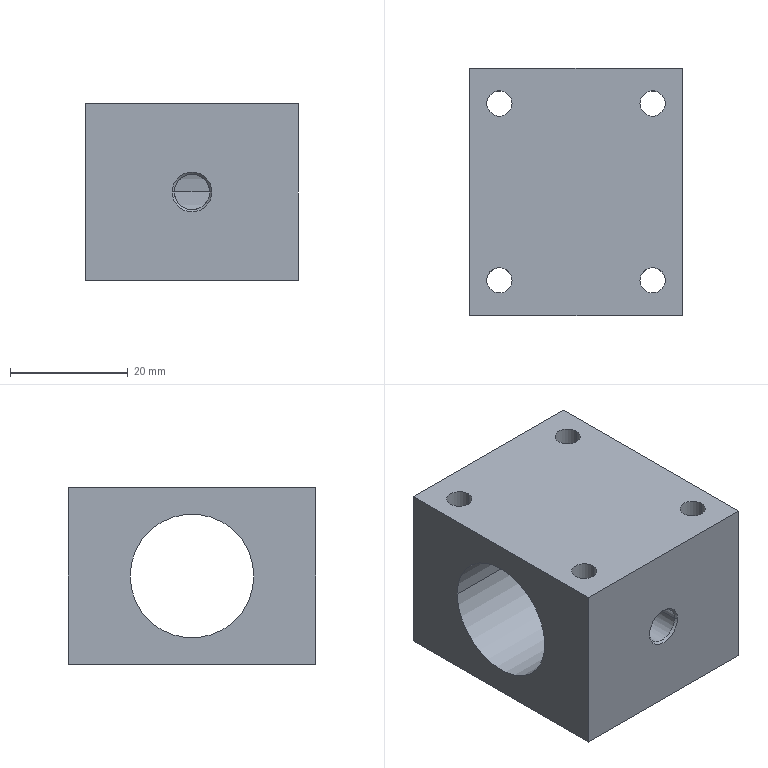Component | SolidWorks | SCLinearBearing-2 | 1 solid | 20 faces | box 36 x 42 x 30 mm | volume 30847 mm3 | cylinder 12 | plane 6 | cone 2 | commonest cylinder face diameters 4.3 x8 6 x2 21 x2
STEP:
#1=COLOUR_RGB('',0.7922,0.8196,0.9333);
#2=FILL_AREA_STYLE_COLOUR('',#1);
#3=FILL_AREA_STYLE('',(#2));
#4=SURFACE_STYLE_FILL_AREA(#3);
#5=SURFACE_SIDE_STYLE('',(#4));
#6=SURFACE_STYLE_USAGE(.BOTH.,#5);
#7=PRESENTATION_STYLE_ASSIGNMENT((#6));
#8=CARTESIAN_POINT('',(8.023,21.078,8.957));
#9=VERTEX_POINT('',#8);
#10=CARTESIAN_POINT('',(7.787,21.078,8.957));
#11=VERTEX_POINT('',#10);
#12=CARTESIAN_POINT('',(7.905,21.078,8.957));
#13=DIRECTION('',(-0.,-1.,-0.));
#14=DIRECTION('',(-1.,0.,0.));
#15=AXIS2_PLACEMENT_3D('',#12,#13,#14);
#16=CIRCLE('',#15,0.1181);
#17=EDGE_CURVE('',#9,#11,#16,.T.);
#18=ORIENTED_EDGE('',*,*,#17,.F.);
#19=CARTESIAN_POINT('',(8.038,21.063,8.957));
#20=VERTEX_POINT('',#19);
#21=CARTESIAN_POINT('',(8.038,21.063,8.957));
#22=DIRECTION('',(0.7071,-0.7071,0.));
#23=VECTOR('',#22,39.37);
#24=LINE('',#21,#23);
#25=EDGE_CURVE('',#9,#20,#24,.T.);
#26=ORIENTED_EDGE('',*,*,#25,.T.);
#27=CARTESIAN_POINT('',(7.772,21.063,8.957));
#28=VERTEX_POINT('',#27);
#29=CARTESIAN_POINT('',(7.905,21.063,8.957));
#30=DIRECTION('',(-0.,-1.,-0.));
#31=DIRECTION('',(-1.,0.,0.));
#32=AXIS2_PLACEMENT_3D('',#29,#30,#31);
#33=CIRCLE('',#32,0.1329);
#34=EDGE_CURVE('',#20,#28,#33,.T.);
#35=ORIENTED_EDGE('',*,*,#34,.T.);
#36=CARTESIAN_POINT('',(7.772,21.063,8.957));
#37=DIRECTION('',(-0.7071,-0.7071,-0.));
#38=VECTOR('',#37,39.37);
#39=LINE('',#36,#38);
#40=EDGE_CURVE('',#11,#28,#39,.T.);
#41=ORIENTED_EDGE('',*,*,#40,.F.);
#42=EDGE_LOOP('',(#18,#26,#35,#41));
#43=FACE_OUTER_BOUND('',#42,.T.);
#44=CARTESIAN_POINT('',(7.905,21.063,8.957));
#45=DIRECTION('',(-0.,-1.,-0.));
#46=DIRECTION('',(-1.,0.,0.));
#47=AXIS2_PLACEMENT_3D('',#44,#45,#46);
#48=CONICAL_SURFACE('',#47,0.1329,0.7854);
#49=ADVANCED_FACE('',(#43),#48,.F.);
#50=CARTESIAN_POINT('',(8.023,21.476,8.957));
#51=VERTEX_POINT('',#50);
#52=CARTESIAN_POINT('',(7.787,21.476,8.957));
#53=VERTEX_POINT('',#52);
#54=CARTESIAN_POINT('',(8.023,21.476,8.957));
#55=CARTESIAN_POINT('',(8.023,21.476,8.964));
#56=CARTESIAN_POINT('',(8.023,21.477,8.972));
#57=CARTESIAN_POINT('',(8.02,21.477,8.988));
#58=CARTESIAN_POINT('',(8.017,21.478,8.995));
#59=CARTESIAN_POINT('',(8.011,21.48,9.009));
#60=CARTESIAN_POINT('',(8.008,21.481,9.016));
#61=CARTESIAN_POINT('',(7.999,21.483,9.029));
#62=CARTESIAN_POINT('',(7.994,21.484,9.035));
#63=CARTESIAN_POINT('',(7.983,21.486,9.046));
#64=CARTESIAN_POINT('',(7.977,21.487,9.051));
#65=CARTESIAN_POINT('',(7.965,21.489,9.059));
#66=CARTESIAN_POINT('',(7.958,21.49,9.063));
#67=CARTESIAN_POINT('',(7.943,21.492,9.069));
#68=CARTESIAN_POINT('',(7.936,21.492,9.071));
#69=CARTESIAN_POINT('',(7.921,21.493,9.074));
#70=CARTESIAN_POINT('',(7.913,21.494,9.075));
#71=CARTESIAN_POINT('',(7.897,21.494,9.075));
#72=CARTESIAN_POINT('',(7.89,21.493,9.074));
#73=CARTESIAN_POINT('',(7.875,21.492,9.071));
#74=CARTESIAN_POINT('',(7.867,21.492,9.069));
#75=CARTESIAN_POINT('',(7.846,21.489,9.06));
#76=CARTESIAN_POINT('',(7.833,21.487,9.051));
#77=CARTESIAN_POINT('',(7.816,21.484,9.035));
#78=CARTESIAN_POINT('',(7.811,21.483,9.029));
#79=CARTESIAN_POINT('',(7.803,21.481,9.016));
#80=CARTESIAN_POINT('',(7.799,21.48,9.009));
#81=CARTESIAN_POINT('',(7.793,21.478,8.995));
#82=CARTESIAN_POINT('',(7.791,21.477,8.987));
#83=CARTESIAN_POINT('',(7.788,21.477,8.972));
#84=CARTESIAN_POINT('',(7.787,21.476,8.965));
#85=CARTESIAN_POINT('',(7.787,21.476,8.957));
#86=B_SPLINE_CURVE_WITH_KNOTS('',3,(#54,#55,#56,#57,#58,#59,#60,#61,#62,#63,#64,#65,#66,#67,#68,#69,#70,#71,#72,#73,#74,#75,#76,#77,#78,#79,#80,#81,#82,#83,#84,#85),.UNSPECIFIED.,.F.,.F.,(4,2,2,2,2,2,2,2,2,2,2,2,2,2,2,4),(0.009429,0.01002,0.01061,0.0112,0.01179,0.01237,0.01296,0.01355,0.01414,0.01473,0.01532,0.0165,0.01709,0.01768,0.01827,0.01885),.UNSPECIFIED.);
#87=EDGE_CURVE('',#51,#53,#86,.T.);
#88=ORIENTED_EDGE('',*,*,#87,.F.);
#89=CARTESIAN_POINT('',(8.023,21.063,8.957));
#90=DIRECTION('',(-0.,-1.,-0.));
#91=VECTOR('',#90,39.37);
#92=LINE('',#89,#91);
#93=EDGE_CURVE('',#51,#9,#92,.T.);
#94=ORIENTED_EDGE('',*,*,#93,.T.);
#95=ORIENTED_EDGE('',*,*,#17,.T.);
#96=CARTESIAN_POINT('',(7.787,21.063,8.957));
#97=DIRECTION('',(-0.,-1.,-0.));
#98=VECTOR('',#97,39.37);
#99=LINE('',#96,#98);
#100=EDGE_CURVE('',#53,#11,#99,.T.);
#101=ORIENTED_EDGE('',*,*,#100,.F.);
#102=EDGE_LOOP('',(#88,#94,#95,#101));
#103=FACE_OUTER_BOUND('',#102,.T.);
#104=CARTESIAN_POINT('',(7.905,21.063,8.957));
#105=DIRECTION('',(-0.,-1.,-0.));
#106=DIRECTION('',(-1.,0.,0.));
#107=AXIS2_PLACEMENT_3D('',#104,#105,#106);
#108=CYLINDRICAL_SURFACE('',#107,0.1181);
#109=ADVANCED_FACE('',(#103),#108,.F.);
#110=CARTESIAN_POINT('',(7.197,22.303,8.957));
#111=VERTEX_POINT('',#110);
#112=CARTESIAN_POINT('',(7.197,21.476,8.957));
#113=VERTEX_POINT('',#112);
#114=CARTESIAN_POINT('',(7.197,21.89,8.957));
#115=DIRECTION('',(1.,-0.,0.));
#116=DIRECTION('',(-0.,-1.,0.));
#117=AXIS2_PLACEMENT_3D('',#114,#115,#116);
#118=CIRCLE('',#117,0.4134);
#119=EDGE_CURVE('',#111,#113,#118,.T.);
#120=ORIENTED_EDGE('',*,*,#119,.F.);
#121=CARTESIAN_POINT('',(8.614,22.303,8.957));
#122=VERTEX_POINT('',#121);
#123=CARTESIAN_POINT('',(8.614,22.303,8.957));
#124=DIRECTION('',(1.,-0.,0.));
#125=VECTOR('',#124,39.37);
#126=LINE('',#123,#125);
#127=EDGE_CURVE('',#111,#122,#126,.T.);
#128=ORIENTED_EDGE('',*,*,#127,.T.);
#129=CARTESIAN_POINT('',(8.614,21.476,8.957));
#130=VERTEX_POINT('',#129);
#131=CARTESIAN_POINT('',(8.614,21.89,8.957));
#132=DIRECTION('',(1.,-0.,0.));
#133=DIRECTION('',(-0.,-1.,0.));
#134=AXIS2_PLACEMENT_3D('',#131,#132,#133);
#135=CIRCLE('',#134,0.4134);
#136=EDGE_CURVE('',#122,#130,#135,.T.);
#137=ORIENTED_EDGE('',*,*,#136,.T.);
#138=CARTESIAN_POINT('',(8.614,21.476,8.957));
#139=DIRECTION('',(1.,-0.,0.));
#140=VECTOR('',#139,39.37);
#141=LINE('',#138,#140);
#142=EDGE_CURVE('',#51,#130,#141,.T.);
#143=ORIENTED_EDGE('',*,*,#142,.F.);
#144=ORIENTED_EDGE('',*,*,#87,.T.);
#145=CARTESIAN_POINT('',(8.614,21.476,8.957));
#146=DIRECTION('',(1.,-0.,0.));
#147=VECTOR('',#146,39.37);
#148=LINE('',#145,#147);
#149=EDGE_CURVE('',#113,#53,#148,.T.);
#150=ORIENTED_EDGE('',*,*,#149,.F.);
#151=EDGE_LOOP('',(#120,#128,#137,#143,#144,#150));
#152=FACE_OUTER_BOUND('',#151,.T.);
#153=CARTESIAN_POINT('',(8.614,21.89,8.957));
#154=DIRECTION('',(1.,-0.,0.));
#155=DIRECTION('',(-0.,-1.,0.));
#156=AXIS2_PLACEMENT_3D('',#153,#154,#155);
#157=CYLINDRICAL_SURFACE('',#156,0.4134);
#158=ADVANCED_FACE('',(#152),#157,.F.);
#159=CARTESIAN_POINT('',(7.478,22.48,8.366));
#160=VERTEX_POINT('',#159);
#161=CARTESIAN_POINT('',(7.309,22.48,8.366));
#162=VERTEX_POINT('',#161);
#163=CARTESIAN_POINT('',(7.393,22.48,8.366));
#164=DIRECTION('',(-0.,-0.,1.));
#165=DIRECTION('',(-1.,0.,0.));
#166=AXIS2_PLACEMENT_3D('',#163,#164,#165);
#167=CIRCLE('',#166,0.08465);
#168=EDGE_CURVE('',#160,#162,#167,.T.);
#169=ORIENTED_EDGE('',*,*,#168,.F.);
#170=CARTESIAN_POINT('',(7.478,22.48,9.547));
#171=VERTEX_POINT('',#170);
#172=CARTESIAN_POINT('',(7.478,22.48,9.547));
#173=DIRECTION('',(-0.,-0.,1.));
#174=VECTOR('',#173,39.37);
#175=LINE('',#172,#174);
#176=EDGE_CURVE('',#160,#171,#175,.T.);
#177=ORIENTED_EDGE('',*,*,#176,.T.);
#178=CARTESIAN_POINT('',(7.309,22.48,9.547));
#179=VERTEX_POINT('',#178);
#180=CARTESIAN_POINT('',(7.393,22.48,9.547));
#181=DIRECTION('',(-0.,-0.,1.));
#182=DIRECTION('',(-1.,0.,0.));
#183=AXIS2_PLACEMENT_3D('',#180,#181,#182);
#184=CIRCLE('',#183,0.08465);
#185=EDGE_CURVE('',#171,#179,#184,.T.);
#186=ORIENTED_EDGE('',*,*,#185,.T.);
#187=CARTESIAN_POINT('',(7.309,22.48,9.547));
#188=DIRECTION('',(-0.,-0.,1.));
#189=VECTOR('',#188,39.37);
#190=LINE('',#187,#189);
#191=EDGE_CURVE('',#162,#179,#190,.T.);
#192=ORIENTED_EDGE('',*,*,#191,.F.);
#193=EDGE_LOOP('',(#169,#177,#186,#192));
#194=FACE_OUTER_BOUND('',#193,.T.);
#195=CARTESIAN_POINT('',(7.393,22.48,9.547));
#196=DIRECTION('',(-0.,-0.,1.));
#197=DIRECTION('',(-1.,0.,0.));
#198=AXIS2_PLACEMENT_3D('',#195,#196,#197);
#199=CYLINDRICAL_SURFACE('',#198,0.08465);
#200=ADVANCED_FACE('',(#194),#199,.F.);
#201=CARTESIAN_POINT('',(8.502,22.48,8.366));
#202=VERTEX_POINT('',#201);
#203=CARTESIAN_POINT('',(8.332,22.48,8.366));
#204=VERTEX_POINT('',#203);
#205=CARTESIAN_POINT('',(8.417,22.48,8.366));
#206=DIRECTION('',(-0.,-0.,1.));
#207=DIRECTION('',(-1.,0.,0.));
#208=AXIS2_PLACEMENT_3D('',#205,#206,#207);
#209=CIRCLE('',#208,0.08465);
#210=EDGE_CURVE('',#202,#204,#209,.T.);
#211=ORIENTED_EDGE('',*,*,#210,.F.);
#212=CARTESIAN_POINT('',(8.502,22.48,9.547));
#213=VERTEX_POINT('',#212);
#214=CARTESIAN_POINT('',(8.502,22.48,9.547));
#215=DIRECTION('',(-0.,-0.,1.));
#216=VECTOR('',#215,39.37);
#217=LINE('',#214,#216);
#218=EDGE_CURVE('',#202,#213,#217,.T.);
#219=ORIENTED_EDGE('',*,*,#218,.T.);
#220=CARTESIAN_POINT('',(8.332,22.48,9.547));
#221=VERTEX_POINT('',#220);
#222=CARTESIAN_POINT('',(8.417,22.48,9.547));
#223=DIRECTION('',(-0.,-0.,1.));
#224=DIRECTION('',(-1.,0.,0.));
#225=AXIS2_PLACEMENT_3D('',#222,#223,#224);
#226=CIRCLE('',#225,0.08465);
#227=EDGE_CURVE('',#213,#221,#226,.T.);
#228=ORIENTED_EDGE('',*,*,#227,.T.);
#229=CARTESIAN_POINT('',(8.332,22.48,9.547));
#230=DIRECTION('',(-0.,-0.,1.));
#231=VECTOR('',#230,39.37);
#232=LINE('',#229,#231);
#233=EDGE_CURVE('',#204,#221,#232,.T.);
#234=ORIENTED_EDGE('',*,*,#233,.F.);
#235=EDGE_LOOP('',(#211,#219,#228,#234));
#236=FACE_OUTER_BOUND('',#235,.T.);
#237=CARTESIAN_POINT('',(8.417,22.48,9.547));
#238=DIRECTION('',(-0.,-0.,1.));
#239=DIRECTION('',(-1.,0.,0.));
#240=AXIS2_PLACEMENT_3D('',#237,#238,#239);
#241=CYLINDRICAL_SURFACE('',#240,0.08465);
#242=ADVANCED_FACE('',(#236),#241,.F.);
#243=CARTESIAN_POINT('',(7.478,21.299,8.366));
#244=VERTEX_POINT('',#243);
#245=CARTESIAN_POINT('',(7.309,21.299,8.366));
#246=VERTEX_POINT('',#245);
#247=CARTESIAN_POINT('',(7.393,21.299,8.366));
#248=DIRECTION('',(-0.,-0.,1.));
#249=DIRECTION('',(-1.,0.,0.));
#250=AXIS2_PLACEMENT_3D('',#247,#248,#249);
#251=CIRCLE('',#250,0.08465);
#252=EDGE_CURVE('',#244,#246,#251,.T.);
#253=ORIENTED_EDGE('',*,*,#252,.F.);
#254=CARTESIAN_POINT('',(7.478,21.299,9.547));
#255=VERTEX_POINT('',#254);
#256=CARTESIAN_POINT('',(7.478,21.299,9.547));
#257=DIRECTION('',(-0.,-0.,1.));
#258=VECTOR('',#257,39.37);
#259=LINE('',#256,#258);
#260=EDGE_CURVE('',#244,#255,#259,.T.);
#261=ORIENTED_EDGE('',*,*,#260,.T.);
#262=CARTESIAN_POINT('',(7.309,21.299,9.547));
#263=VERTEX_POINT('',#262);
#264=CARTESIAN_POINT('',(7.393,21.299,9.547));
#265=DIRECTION('',(-0.,-0.,1.));
#266=DIRECTION('',(-1.,0.,0.));
#267=AXIS2_PLACEMENT_3D('',#264,#265,#266);
#268=CIRCLE('',#267,0.08465);
#269=EDGE_CURVE('',#255,#263,#268,.T.);
#270=ORIENTED_EDGE('',*,*,#269,.T.);
#271=CARTESIAN_POINT('',(7.309,21.299,9.547));
#272=DIRECTION('',(-0.,-0.,1.));
#273=VECTOR('',#272,39.37);
#274=LINE('',#271,#273);
#275=EDGE_CURVE('',#246,#263,#274,.T.);
#276=ORIENTED_EDGE('',*,*,#275,.F.);
#277=EDGE_LOOP('',(#253,#261,#270,#276));
#278=FACE_OUTER_BOUND('',#277,.T.);
#279=CARTESIAN_POINT('',(7.393,21.299,9.547));
#280=DIRECTION('',(-0.,-0.,1.));
#281=DIRECTION('',(-1.,0.,0.));
#282=AXIS2_PLACEMENT_3D('',#279,#280,#281);
#283=CYLINDRICAL_SURFACE('',#282,0.08465);
#284=ADVANCED_FACE('',(#278),#283,.F.);
#285=CARTESIAN_POINT('',(8.502,21.299,8.366));
#286=VERTEX_POINT('',#285);
#287=CARTESIAN_POINT('',(8.332,21.299,8.366));
#288=VERTEX_POINT('',#287);
#289=CARTESIAN_POINT('',(8.417,21.299,8.366));
#290=DIRECTION('',(-0.,-0.,1.));
#291=DIRECTION('',(-1.,0.,0.));
#292=AXIS2_PLACEMENT_3D('',#289,#290,#291);
#293=CIRCLE('',#292,0.08465);
#294=EDGE_CURVE('',#286,#288,#293,.T.);
#295=ORIENTED_EDGE('',*,*,#294,.F.);
#296=CARTESIAN_POINT('',(8.502,21.299,9.547));
#297=VERTEX_POINT('',#296);
#298=CARTESIAN_POINT('',(8.502,21.299,9.547));
#299=DIRECTION('',(-0.,-0.,1.));
#300=VECTOR('',#299,39.37);
#301=LINE('',#298,#300);
#302=EDGE_CURVE('',#286,#297,#301,.T.);
#303=ORIENTED_EDGE('',*,*,#302,.T.);
#304=CARTESIAN_POINT('',(8.332,21.299,9.547));
#305=VERTEX_POINT('',#304);
#306=CARTESIAN_POINT('',(8.417,21.299,9.547));
#307=DIRECTION('',(-0.,-0.,1.));
#308=DIRECTION('',(-1.,0.,0.));
#309=AXIS2_PLACEMENT_3D('',#306,#307,#308);
#310=CIRCLE('',#309,0.08465);
#311=EDGE_CURVE('',#297,#305,#310,.T.);
#312=ORIENTED_EDGE('',*,*,#311,.T.);
#313=CARTESIAN_POINT('',(8.332,21.299,9.547));
#314=DIRECTION('',(-0.,-0.,1.));
#315=VECTOR('',#314,39.37);
#316=LINE('',#313,#315);
#317=EDGE_CURVE('',#288,#305,#316,.T.);
#318=ORIENTED_EDGE('',*,*,#317,.F.);
#319=EDGE_LOOP('',(#295,#303,#312,#318));
#320=FACE_OUTER_BOUND('',#319,.T.);
#321=CARTESIAN_POINT('',(8.417,21.299,9.547));
#322=DIRECTION('',(-0.,-0.,1.));
#323=DIRECTION('',(-1.,0.,0.));
#324=AXIS2_PLACEMENT_3D('',#321,#322,#323);
#325=CYLINDRICAL_SURFACE('',#324,0.08465);
#326=ADVANCED_FACE('',(#320),#325,.F.);
#327=CARTESIAN_POINT('',(7.197,22.717,9.547));
#328=VERTEX_POINT('',#327);
#329=CARTESIAN_POINT('',(7.197,21.063,9.547));
#330=VERTEX_POINT('',#329);
#331=CARTESIAN_POINT('',(7.197,22.717,9.547));
#332=DIRECTION('',(-0.,-1.,-0.));
#333=VECTOR('',#332,39.37);
#334=LINE('',#331,#333);
#335=EDGE_CURVE('',#328,#330,#334,.T.);
#336=ORIENTED_EDGE('',*,*,#335,.F.);
#337=CARTESIAN_POINT('',(7.197,22.717,8.366));
#338=VERTEX_POINT('',#337);
#339=CARTESIAN_POINT('',(7.197,22.717,8.366));
#340=DIRECTION('',(-0.,-0.,1.));
#341=VECTOR('',#340,39.37);
#342=LINE('',#339,#341);
#343=EDGE_CURVE('',#338,#328,#342,.T.);
#344=ORIENTED_EDGE('',*,*,#343,.F.);
#345=CARTESIAN_POINT('',(7.197,21.063,8.366));
#346=VERTEX_POINT('',#345);
#347=CARTESIAN_POINT('',(7.197,22.717,8.366));
#348=DIRECTION('',(-0.,-1.,-0.));
#349=VECTOR('',#348,39.37);
#350=LINE('',#347,#349);
#351=EDGE_CURVE('',#338,#346,#350,.T.);
#352=ORIENTED_EDGE('',*,*,#351,.T.);
#353=CARTESIAN_POINT('',(7.197,21.063,8.366));
#354=DIRECTION('',(-0.,-0.,1.));
#355=VECTOR('',#354,39.37);
#356=LINE('',#353,#355);
#357=EDGE_CURVE('',#346,#330,#356,.T.);
#358=ORIENTED_EDGE('',*,*,#357,.T.);
#359=EDGE_LOOP('',(#336,#344,#352,#358));
#360=FACE_OUTER_BOUND('',#359,.T.);
#361=CARTESIAN_POINT('',(7.197,21.89,8.957));
#362=DIRECTION('',(1.,-0.,0.));
#363=DIRECTION('',(-0.,-1.,0.));
#364=AXIS2_PLACEMENT_3D('',#361,#362,#363);
#365=CIRCLE('',#364,0.4134);
#366=EDGE_CURVE('',#113,#111,#365,.T.);
#367=ORIENTED_EDGE('',*,*,#366,.T.);
#368=ORIENTED_EDGE('',*,*,#119,.T.);
#369=EDGE_LOOP('',(#367,#368));
#370=FACE_BOUND('',#369,.T.);
#371=CARTESIAN_POINT('',(7.197,22.717,8.366));
#372=DIRECTION('',(-1.,0.,-0.));
#373=DIRECTION('',(0.,1.,0.));
#374=AXIS2_PLACEMENT_3D('',#371,#372,#373);
#375=PLANE('',#374);
#376=ADVANCED_FACE('',(#360,#370),#375,.T.);
#377=CARTESIAN_POINT('',(7.905,21.063,8.957));
#378=DIRECTION('',(-0.,-1.,-0.));
#379=DIRECTION('',(-1.,0.,0.));
#380=AXIS2_PLACEMENT_3D('',#377,#378,#379);
#381=CIRCLE('',#380,0.1329);
#382=EDGE_CURVE('',#28,#20,#381,.T.);
#383=ORIENTED_EDGE('',*,*,#382,.F.);
#384=ORIENTED_EDGE('',*,*,#34,.F.);
#385=EDGE_LOOP('',(#383,#384));
#386=FACE_BOUND('',#385,.T.);
#387=CARTESIAN_POINT('',(8.614,21.063,9.547));
#388=VERTEX_POINT('',#387);
#389=CARTESIAN_POINT('',(7.197,21.063,9.547));
#390=DIRECTION('',(1.,-0.,0.));
#391=VECTOR('',#390,39.37);
#392=LINE('',#389,#391);
#393=EDGE_CURVE('',#330,#388,#392,.T.);
#394=ORIENTED_EDGE('',*,*,#393,.F.);
#395=ORIENTED_EDGE('',*,*,#357,.F.);
#396=CARTESIAN_POINT('',(8.614,21.063,8.366));
#397=VERTEX_POINT('',#396);
#398=CARTESIAN_POINT('',(7.197,21.063,8.366));
#399=DIRECTION('',(1.,-0.,0.));
#400=VECTOR('',#399,39.37);
#401=LINE('',#398,#400);
#402=EDGE_CURVE('',#346,#397,#401,.T.);
#403=ORIENTED_EDGE('',*,*,#402,.T.);
#404=CARTESIAN_POINT('',(8.614,21.063,8.366));
#405=DIRECTION('',(-0.,-0.,1.));
#406=VECTOR('',#405,39.37);
#407=LINE('',#404,#406);
#408=EDGE_CURVE('',#397,#388,#407,.T.);
#409=ORIENTED_EDGE('',*,*,#408,.T.);
#410=EDGE_LOOP('',(#394,#395,#403,#409));
#411=FACE_OUTER_BOUND('',#410,.T.);
#412=CARTESIAN_POINT('',(7.197,21.063,8.366));
#413=DIRECTION('',(-0.,-1.,-0.));
#414=DIRECTION('',(-1.,0.,-0.));
#415=AXIS2_PLACEMENT_3D('',#412,#413,#414);
#416=PLANE('',#415);
#417=ADVANCED_FACE('',(#386,#411),#416,.T.);
#418=CARTESIAN_POINT('',(8.614,22.717,9.547));
#419=VERTEX_POINT('',#418);
#420=CARTESIAN_POINT('',(8.614,22.717,9.547));
#421=DIRECTION('',(-1.,0.,-0.));
#422=VECTOR('',#421,39.37);
#423=LINE('',#420,#422);
#424=EDGE_CURVE('',#419,#328,#423,.T.);
#425=ORIENTED_EDGE('',*,*,#424,.F.);
#426=CARTESIAN_POINT('',(8.614,22.717,8.366));
#427=VERTEX_POINT('',#426);
#428=CARTESIAN_POINT('',(8.614,22.717,8.366));
#429=DIRECTION('',(-0.,-0.,1.));
#430=VECTOR('',#429,39.37);
#431=LINE('',#428,#430);
#432=EDGE_CURVE('',#427,#419,#431,.T.);
#433=ORIENTED_EDGE('',*,*,#432,.F.);
#434=CARTESIAN_POINT('',(8.614,22.717,8.366));
#435=DIRECTION('',(-1.,0.,-0.));
#436=VECTOR('',#435,39.37);
#437=LINE('',#434,#436);
#438=EDGE_CURVE('',#427,#338,#437,.T.);
#439=ORIENTED_EDGE('',*,*,#438,.T.);
#440=ORIENTED_EDGE('',*,*,#343,.T.);
#441=EDGE_LOOP('',(#425,#433,#439,#440));
#442=FACE_OUTER_BOUND('',#441,.T.);
#443=CARTESIAN_POINT('',(8.614,22.717,8.366));
#444=DIRECTION('',(0.,1.,0.));
#445=DIRECTION('',(1.,-0.,0.));
#446=AXIS2_PLACEMENT_3D('',#443,#444,#445);
#447=PLANE('',#446);
#448=ADVANCED_FACE('',(#442),#447,.T.);
#449=CARTESIAN_POINT('',(8.614,21.89,8.957));
#450=DIRECTION('',(1.,-0.,0.));
#451=DIRECTION('',(-0.,-1.,0.));
#452=AXIS2_PLACEMENT_3D('',#449,#450,#451);
#453=CIRCLE('',#452,0.4134);
#454=EDGE_CURVE('',#130,#122,#453,.T.);
#455=ORIENTED_EDGE('',*,*,#454,.F.);
#456=ORIENTED_EDGE('',*,*,#136,.F.);
#457=EDGE_LOOP('',(#455,#456));
#458=FACE_BOUND('',#457,.T.);
#459=CARTESIAN_POINT('',(8.614,21.063,9.547));
#460=DIRECTION('',(0.,1.,0.));
#461=VECTOR('',#460,39.37);
#462=LINE('',#459,#461);
#463=EDGE_CURVE('',#388,#419,#462,.T.);
#464=ORIENTED_EDGE('',*,*,#463,.F.);
#465=ORIENTED_EDGE('',*,*,#408,.F.);
#466=CARTESIAN_POINT('',(8.614,21.063,8.366));
#467=DIRECTION('',(0.,1.,0.));
#468=VECTOR('',#467,39.37);
#469=LINE('',#466,#468);
#470=EDGE_CURVE('',#397,#427,#469,.T.);
#471=ORIENTED_EDGE('',*,*,#470,.T.);
#472=ORIENTED_EDGE('',*,*,#432,.T.);
#473=EDGE_LOOP('',(#464,#465,#471,#472));
#474=FACE_OUTER_BOUND('',#473,.T.);
#475=CARTESIAN_POINT('',(8.614,21.063,8.366));
#476=DIRECTION('',(1.,-0.,0.));
#477=DIRECTION('',(-0.,-1.,-0.));
#478=AXIS2_PLACEMENT_3D('',#475,#476,#477);
#479=PLANE('',#478);
#480=ADVANCED_FACE('',(#458,#474),#479,.T.);
#481=CARTESIAN_POINT('',(7.393,22.48,8.366));
#482=DIRECTION('',(-0.,-0.,1.));
#483=DIRECTION('',(-1.,0.,0.));
#484=AXIS2_PLACEMENT_3D('',#481,#482,#483);
#485=CIRCLE('',#484,0.08465);
#486=EDGE_CURVE('',#162,#160,#485,.T.);
#487=ORIENTED_EDGE('',*,*,#486,.T.);
#488=ORIENTED_EDGE('',*,*,#168,.T.);
#489=EDGE_LOOP('',(#487,#488));
#490=FACE_BOUND('',#489,.T.);
#491=CARTESIAN_POINT('',(8.417,22.48,8.366));
#492=DIRECTION('',(-0.,-0.,1.));
#493=DIRECTION('',(-1.,0.,0.));
#494=AXIS2_PLACEMENT_3D('',#491,#492,#493);
#495=CIRCLE('',#494,0.08465);
#496=EDGE_CURVE('',#204,#202,#495,.T.);
#497=ORIENTED_EDGE('',*,*,#496,.T.);
#498=ORIENTED_EDGE('',*,*,#210,.T.);
#499=EDGE_LOOP('',(#497,#498));
#500=FACE_BOUND('',#499,.T.);
#501=CARTESIAN_POINT('',(7.393,21.299,8.366));
#502=DIRECTION('',(-0.,-0.,1.));
#503=DIRECTION('',(-1.,0.,0.));
#504=AXIS2_PLACEMENT_3D('',#501,#502,#503);
#505=CIRCLE('',#504,0.08465);
#506=EDGE_CURVE('',#246,#244,#505,.T.);
#507=ORIENTED_EDGE('',*,*,#506,.T.);
#508=ORIENTED_EDGE('',*,*,#252,.T.);
#509=EDGE_LOOP('',(#507,#508));
#510=FACE_BOUND('',#509,.T.);
#511=CARTESIAN_POINT('',(8.417,21.299,8.366));
#512=DIRECTION('',(-0.,-0.,1.));
#513=DIRECTION('',(-1.,0.,0.));
#514=AXIS2_PLACEMENT_3D('',#511,#512,#513);
#515=CIRCLE('',#514,0.08465);
#516=EDGE_CURVE('',#288,#286,#515,.T.);
#517=ORIENTED_EDGE('',*,*,#516,.T.);
#518=ORIENTED_EDGE('',*,*,#294,.T.);
#519=EDGE_LOOP('',(#517,#518));
#520=FACE_BOUND('',#519,.T.);
#521=ORIENTED_EDGE('',*,*,#402,.F.);
#522=ORIENTED_EDGE('',*,*,#351,.F.);
#523=ORIENTED_EDGE('',*,*,#438,.F.);
#524=ORIENTED_EDGE('',*,*,#470,.F.);
#525=EDGE_LOOP('',(#521,#522,#523,#524));
#526=FACE_OUTER_BOUND('',#525,.T.);
#527=CARTESIAN_POINT('',(7.905,21.89,8.366));
#528=DIRECTION('',(-0.,-0.,1.));
#529=DIRECTION('',(-1.,0.,-0.));
#530=AXIS2_PLACEMENT_3D('',#527,#528,#529);
#531=PLANE('',#530);
#532=ADVANCED_FACE('',(#490,#500,#510,#520,#526),#531,.F.);
#533=CARTESIAN_POINT('',(7.393,22.48,9.547));
#534=DIRECTION('',(-0.,-0.,1.));
#535=DIRECTION('',(-1.,0.,0.));
#536=AXIS2_PLACEMENT_3D('',#533,#534,#535);
#537=CIRCLE('',#536,0.08465);
#538=EDGE_CURVE('',#179,#171,#537,.T.);
#539=ORIENTED_EDGE('',*,*,#538,.F.);
#540=ORIENTED_EDGE('',*,*,#185,.F.);
#541=EDGE_LOOP('',(#539,#540));
#542=FACE_BOUND('',#541,.T.);
#543=CARTESIAN_POINT('',(8.417,22.48,9.547));
#544=DIRECTION('',(-0.,-0.,1.));
#545=DIRECTION('',(-1.,0.,0.));
#546=AXIS2_PLACEMENT_3D('',#543,#544,#545);
#547=CIRCLE('',#546,0.08465);
#548=EDGE_CURVE('',#221,#213,#547,.T.);
#549=ORIENTED_EDGE('',*,*,#548,.F.);
#550=ORIENTED_EDGE('',*,*,#227,.F.);
#551=EDGE_LOOP('',(#549,#550));
#552=FACE_BOUND('',#551,.T.);
#553=CARTESIAN_POINT('',(7.393,21.299,9.547));
#554=DIRECTION('',(-0.,-0.,1.));
#555=DIRECTION('',(-1.,0.,0.));
#556=AXIS2_PLACEMENT_3D('',#553,#554,#555);
#557=CIRCLE('',#556,0.08465);
#558=EDGE_CURVE('',#263,#255,#557,.T.);
#559=ORIENTED_EDGE('',*,*,#558,.F.);
#560=ORIENTED_EDGE('',*,*,#269,.F.);
#561=EDGE_LOOP('',(#559,#560));
#562=FACE_BOUND('',#561,.T.);
#563=CARTESIAN_POINT('',(8.417,21.299,9.547));
#564=DIRECTION('',(-0.,-0.,1.));
#565=DIRECTION('',(-1.,0.,0.));
#566=AXIS2_PLACEMENT_3D('',#563,#564,#565);
#567=CIRCLE('',#566,0.08465);
#568=EDGE_CURVE('',#305,#297,#567,.T.);
#569=ORIENTED_EDGE('',*,*,#568,.F.);
#570=ORIENTED_EDGE('',*,*,#311,.F.);
#571=EDGE_LOOP('',(#569,#570));
#572=FACE_BOUND('',#571,.T.);
#573=ORIENTED_EDGE('',*,*,#393,.T.);
#574=ORIENTED_EDGE('',*,*,#463,.T.);
#575=ORIENTED_EDGE('',*,*,#424,.T.);
#576=ORIENTED_EDGE('',*,*,#335,.T.);
#577=EDGE_LOOP('',(#573,#574,#575,#576));
#578=FACE_OUTER_BOUND('',#577,.T.);
#579=CARTESIAN_POINT('',(7.905,21.89,9.547));
#580=DIRECTION('',(-0.,-0.,1.));
#581=DIRECTION('',(-1.,0.,-0.));
#582=AXIS2_PLACEMENT_3D('',#579,#580,#581);
#583=PLANE('',#582);
#584=ADVANCED_FACE('',(#542,#552,#562,#572,#578),#583,.T.);
#585=ORIENTED_EDGE('',*,*,#302,.F.);
#586=ORIENTED_EDGE('',*,*,#516,.F.);
#587=ORIENTED_EDGE('',*,*,#317,.T.);
#588=ORIENTED_EDGE('',*,*,#568,.T.);
#589=EDGE_LOOP('',(#585,#586,#587,#588));
#590=FACE_OUTER_BOUND('',#589,.T.);
#591=CARTESIAN_POINT('',(8.417,21.299,9.547));
#592=DIRECTION('',(-0.,-0.,1.));
#593=DIRECTION('',(-1.,0.,0.));
#594=AXIS2_PLACEMENT_3D('',#591,#592,#593);
#595=CYLINDRICAL_SURFACE('',#594,0.08465);
#596=ADVANCED_FACE('',(#590),#595,.F.);
#597=ORIENTED_EDGE('',*,*,#260,.F.);
#598=ORIENTED_EDGE('',*,*,#506,.F.);
#599=ORIENTED_EDGE('',*,*,#275,.T.);
#600=ORIENTED_EDGE('',*,*,#558,.T.);
#601=EDGE_LOOP('',(#597,#598,#599,#600));
#602=FACE_OUTER_BOUND('',#601,.T.);
#603=CARTESIAN_POINT('',(7.393,21.299,9.547));
#604=DIRECTION('',(-0.,-0.,1.));
#605=DIRECTION('',(-1.,0.,0.));
#606=AXIS2_PLACEMENT_3D('',#603,#604,#605);
#607=CYLINDRICAL_SURFACE('',#606,0.08465);
#608=ADVANCED_FACE('',(#602),#607,.F.);
#609=ORIENTED_EDGE('',*,*,#218,.F.);
#610=ORIENTED_EDGE('',*,*,#496,.F.);
#611=ORIENTED_EDGE('',*,*,#233,.T.);
#612=ORIENTED_EDGE('',*,*,#548,.T.);
#613=EDGE_LOOP('',(#609,#610,#611,#612));
#614=FACE_OUTER_BOUND('',#613,.T.);
#615=CARTESIAN_POINT('',(8.417,22.48,9.547));
#616=DIRECTION('',(-0.,-0.,1.));
#617=DIRECTION('',(-1.,0.,0.));
#618=AXIS2_PLACEMENT_3D('',#615,#616,#617);
#619=CYLINDRICAL_SURFACE('',#618,0.08465);
#620=ADVANCED_FACE('',(#614),#619,.F.);
#621=ORIENTED_EDGE('',*,*,#176,.F.);
#622=ORIENTED_EDGE('',*,*,#486,.F.);
#623=ORIENTED_EDGE('',*,*,#191,.T.);
#624=ORIENTED_EDGE('',*,*,#538,.T.);
#625=EDGE_LOOP('',(#621,#622,#623,#624));
#626=FACE_OUTER_BOUND('',#625,.T.);
#627=CARTESIAN_POINT('',(7.393,22.48,9.547));
#628=DIRECTION('',(-0.,-0.,1.));
#629=DIRECTION('',(-1.,0.,0.));
#630=AXIS2_PLACEMENT_3D('',#627,#628,#629);
#631=CYLINDRICAL_SURFACE('',#630,0.08465);
#632=ADVANCED_FACE('',(#626),#631,.F.);
#633=ORIENTED_EDGE('',*,*,#127,.F.);
#634=ORIENTED_EDGE('',*,*,#366,.F.);
#635=ORIENTED_EDGE('',*,*,#149,.T.);
#636=CARTESIAN_POINT('',(7.787,21.476,8.957));
#637=CARTESIAN_POINT('',(7.787,21.476,8.949));
#638=CARTESIAN_POINT('',(7.788,21.477,8.941));
#639=CARTESIAN_POINT('',(7.791,21.477,8.926));
#640=CARTESIAN_POINT('',(7.793,21.478,8.918));
#641=CARTESIAN_POINT('',(7.799,21.48,8.904));
#642=CARTESIAN_POINT('',(7.803,21.481,8.897));
#643=CARTESIAN_POINT('',(7.811,21.483,8.885));
#644=CARTESIAN_POINT('',(7.816,21.484,8.879));
#645=CARTESIAN_POINT('',(7.833,21.487,8.862));
#646=CARTESIAN_POINT('',(7.846,21.489,8.854));
#647=CARTESIAN_POINT('',(7.867,21.492,8.845));
#648=CARTESIAN_POINT('',(7.874,21.492,8.842));
#649=CARTESIAN_POINT('',(7.89,21.493,8.839));
#650=CARTESIAN_POINT('',(7.897,21.494,8.839));
#651=CARTESIAN_POINT('',(7.913,21.494,8.839));
#652=CARTESIAN_POINT('',(7.921,21.493,8.839));
#653=CARTESIAN_POINT('',(7.936,21.492,8.842));
#654=CARTESIAN_POINT('',(7.943,21.492,8.845));
#655=CARTESIAN_POINT('',(7.965,21.489,8.854));
#656=CARTESIAN_POINT('',(7.978,21.487,8.862));
#657=CARTESIAN_POINT('',(7.994,21.484,8.879));
#658=CARTESIAN_POINT('',(7.999,21.483,8.885));
#659=CARTESIAN_POINT('',(8.008,21.481,8.897));
#660=CARTESIAN_POINT('',(8.011,21.48,8.904));
#661=CARTESIAN_POINT('',(8.017,21.478,8.919));
#662=CARTESIAN_POINT('',(8.02,21.477,8.926));
#663=CARTESIAN_POINT('',(8.023,21.477,8.941));
#664=CARTESIAN_POINT('',(8.023,21.476,8.949));
#665=CARTESIAN_POINT('',(8.023,21.476,8.957));
#666=B_SPLINE_CURVE_WITH_KNOTS('',3,(#636,#637,#638,#639,#640,#641,#642,#643,#644,#645,#646,#647,#648,#649,#650,#651,#652,#653,#654,#655,#656,#657,#658,#659,#660,#661,#662,#663,#664,#665),.UNSPECIFIED.,.F.,.F.,(4,2,2,2,2,2,2,2,2,2,2,2,2,2,4),(0.,0.0005893,0.001179,0.001768,0.002357,0.003536,0.004125,0.004714,0.005304,0.005893,0.007072,0.007661,0.00825,0.008839,0.009429),.UNSPECIFIED.);
#667=EDGE_CURVE('',#53,#51,#666,.T.);
#668=ORIENTED_EDGE('',*,*,#667,.T.);
#669=ORIENTED_EDGE('',*,*,#142,.T.);
#670=ORIENTED_EDGE('',*,*,#454,.T.);
#671=EDGE_LOOP('',(#633,#634,#635,#668,#669,#670));
#672=FACE_OUTER_BOUND('',#671,.T.);
#673=CARTESIAN_POINT('',(8.614,21.89,8.957));
#674=DIRECTION('',(1.,-0.,0.));
#675=DIRECTION('',(-0.,-1.,0.));
#676=AXIS2_PLACEMENT_3D('',#673,#674,#675);
#677=CYLINDRICAL_SURFACE('',#676,0.4134);
#678=ADVANCED_FACE('',(#672),#677,.F.);
#679=ORIENTED_EDGE('',*,*,#93,.F.);
#680=ORIENTED_EDGE('',*,*,#667,.F.);
#681=ORIENTED_EDGE('',*,*,#100,.T.);
#682=CARTESIAN_POINT('',(7.905,21.078,8.957));
#683=DIRECTION('',(-0.,-1.,-0.));
#684=DIRECTION('',(-1.,0.,0.));
#685=AXIS2_PLACEMENT_3D('',#682,#683,#684);
#686=CIRCLE('',#685,0.1181);
#687=EDGE_CURVE('',#11,#9,#686,.T.);
#688=ORIENTED_EDGE('',*,*,#687,.T.);
#689=EDGE_LOOP('',(#679,#680,#681,#688));
#690=FACE_OUTER_BOUND('',#689,.T.);
#691=CARTESIAN_POINT('',(7.905,21.063,8.957));
#692=DIRECTION('',(-0.,-1.,-0.));
#693=DIRECTION('',(-1.,0.,0.));
#694=AXIS2_PLACEMENT_3D('',#691,#692,#693);
#695=CYLINDRICAL_SURFACE('',#694,0.1181);
#696=ADVANCED_FACE('',(#690),#695,.F.);
#697=ORIENTED_EDGE('',*,*,#25,.F.);
#698=ORIENTED_EDGE('',*,*,#687,.F.);
#699=ORIENTED_EDGE('',*,*,#40,.T.);
#700=ORIENTED_EDGE('',*,*,#382,.T.);
#701=EDGE_LOOP('',(#697,#698,#699,#700));
#702=FACE_OUTER_BOUND('',#701,.T.);
#703=CARTESIAN_POINT('',(7.905,21.063,8.957));
#704=DIRECTION('',(-0.,-1.,-0.));
#705=DIRECTION('',(-1.,0.,0.));
#706=AXIS2_PLACEMENT_3D('',#703,#704,#705);
#707=CONICAL_SURFACE('',#706,0.1329,0.7854);
#708=ADVANCED_FACE('',(#702),#707,.F.);
#709=CLOSED_SHELL('',(#49,#109,#158,#200,#242,#284,#326,#376,#417,#448,#480,#532,#584,#596,#608,#620,#632,#678,#696,#708));
#710=MANIFOLD_SOLID_BREP('',#709);
#711=STYLED_ITEM('',(#7),#710);
#712=PRESENTATION_LAYER_ASSIGNMENT('','',(#711));
#713=CARTESIAN_POINT('',(0.,0.,0.));
#714=DIRECTION('',(0.,0.,1.));
#715=DIRECTION('',(1.,0.,0.));
#716=AXIS2_PLACEMENT_3D('',#713,#714,#715);
#717=(LENGTH_UNIT()NAMED_UNIT(*)SI_UNIT($,.METRE.));
#718=LENGTH_MEASURE_WITH_UNIT(LENGTH_MEASURE(0.0254),#717);
#719=DIMENSIONAL_EXPONENTS(1.,0.,0.,0.,0.,0.,0.);
#720=(CONVERSION_BASED_UNIT('',#718)LENGTH_UNIT()NAMED_UNIT(#719));
#721=UNCERTAINTY_MEASURE_WITH_UNIT(LENGTH_MEASURE(0.00001),#720,'','');
#722=(NAMED_UNIT(*)PLANE_ANGLE_UNIT()SI_UNIT($,.RADIAN.));
#723=(NAMED_UNIT(*)SI_UNIT($,.STERADIAN.)SOLID_ANGLE_UNIT());
#724=(GEOMETRIC_REPRESENTATION_CONTEXT(3)GLOBAL_UNCERTAINTY_ASSIGNED_CONTEXT((#721))GLOBAL_UNIT_ASSIGNED_CONTEXT((#720,#722,#723))REPRESENTATION_CONTEXT('',''));
#725=ADVANCED_BREP_SHAPE_REPRESENTATION('',(#710,#716),#724);
#726=(LENGTH_UNIT()NAMED_UNIT(*)SI_UNIT($,.METRE.));
#727=LENGTH_MEASURE_WITH_UNIT(LENGTH_MEASURE(0.0254),#726);
#728=DIMENSIONAL_EXPONENTS(1.,0.,0.,0.,0.,0.,0.);
#729=(CONVERSION_BASED_UNIT('',#727)LENGTH_UNIT()NAMED_UNIT(#728));
#730=UNCERTAINTY_MEASURE_WITH_UNIT(LENGTH_MEASURE(0.00001),#729,'','');
#731=(NAMED_UNIT(*)PLANE_ANGLE_UNIT()SI_UNIT($,.RADIAN.));
#732=(NAMED_UNIT(*)SI_UNIT($,.STERADIAN.)SOLID_ANGLE_UNIT());
#733=(GEOMETRIC_REPRESENTATION_CONTEXT(3)GLOBAL_UNCERTAINTY_ASSIGNED_CONTEXT((#730))GLOBAL_UNIT_ASSIGNED_CONTEXT((#729,#731,#732))REPRESENTATION_CONTEXT('',''));
#734=MECHANICAL_DESIGN_GEOMETRIC_PRESENTATION_REPRESENTATION('',(#711),#733);